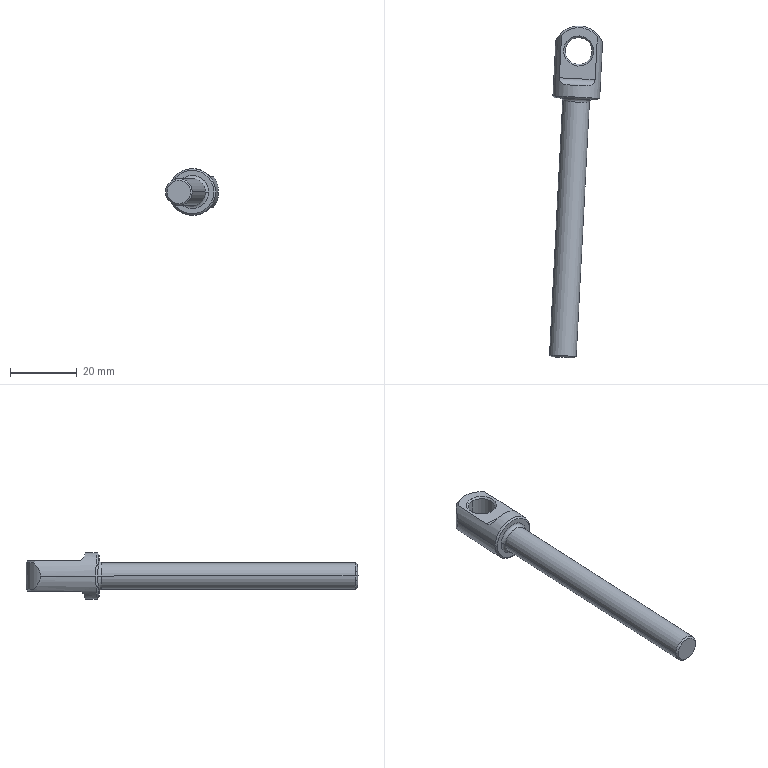Component | SolidWorks | CylinderAxis-1 | 1 solid | 28 faces | box 15.86 x 99.37 x 14 mm | volume 6011 mm3 | cone 11 | cylinder 9 | plane 6 | torus 2 | commonest cylinder face diameters 8 x4 14 x2 4 x2 15 x1
STEP:
#1=COLOUR_RGB('',0.7922,0.8196,0.9333);
#2=FILL_AREA_STYLE_COLOUR('',#1);
#3=FILL_AREA_STYLE('',(#2));
#4=SURFACE_STYLE_FILL_AREA(#3);
#5=SURFACE_SIDE_STYLE('',(#4));
#6=SURFACE_STYLE_USAGE(.BOTH.,#5);
#7=PRESENTATION_STYLE_ASSIGNMENT((#6));
#8=CARTESIAN_POINT('',(4.691,-4.191,6.691));
#9=VERTEX_POINT('',#8);
#10=CARTESIAN_POINT('',(4.415,-4.176,6.691));
#11=VERTEX_POINT('',#10);
#12=CARTESIAN_POINT('',(4.553,-4.184,6.691));
#13=DIRECTION('',(-0.0519,-0.9987,0.));
#14=DIRECTION('',(0.9987,-0.0519,0.));
#15=AXIS2_PLACEMENT_3D('',#12,#13,#14);
#16=CIRCLE('',#15,0.1378);
#17=EDGE_CURVE('',#9,#11,#16,.T.);
#18=ORIENTED_EDGE('',*,*,#17,.F.);
#19=CARTESIAN_POINT('',(4.711,-4.172,6.691));
#20=VERTEX_POINT('',#19);
#21=CARTESIAN_POINT('',(4.691,-4.191,6.691));
#22=DIRECTION('',(0.7429,0.6695,0.));
#23=VECTOR('',#22,39.37);
#24=LINE('',#21,#23);
#25=EDGE_CURVE('',#9,#20,#24,.T.);
#26=ORIENTED_EDGE('',*,*,#25,.T.);
#27=CARTESIAN_POINT('',(4.397,-4.156,6.691));
#28=VERTEX_POINT('',#27);
#29=CARTESIAN_POINT('',(4.554,-4.164,6.691));
#30=DIRECTION('',(0.0519,0.9987,-0.));
#31=DIRECTION('',(0.9987,-0.0519,0.));
#32=AXIS2_PLACEMENT_3D('',#29,#30,#31);
#33=CIRCLE('',#32,0.1575);
#34=EDGE_CURVE('',#28,#20,#33,.T.);
#35=ORIENTED_EDGE('',*,*,#34,.F.);
#36=CARTESIAN_POINT('',(4.415,-4.176,6.691));
#37=DIRECTION('',(-0.6695,0.7429,-0.));
#38=VECTOR('',#37,39.37);
#39=LINE('',#36,#38);
#40=EDGE_CURVE('',#11,#28,#39,.T.);
#41=ORIENTED_EDGE('',*,*,#40,.F.);
#42=EDGE_LOOP('',(#18,#26,#35,#41));
#43=FACE_OUTER_BOUND('',#42,.T.);
#44=CARTESIAN_POINT('',(4.553,-4.184,6.691));
#45=DIRECTION('',(0.0519,0.9987,-0.));
#46=DIRECTION('',(-0.9987,0.0519,0.));
#47=AXIS2_PLACEMENT_3D('',#44,#45,#46);
#48=CONICAL_SURFACE('',#47,0.1378,0.7854);
#49=ADVANCED_FACE('',(#43),#48,.T.);
#50=CARTESIAN_POINT('',(4.755,-0.2988,6.514));
#51=VERTEX_POINT('',#50);
#52=CARTESIAN_POINT('',(4.961,-0.408,6.514));
#53=VERTEX_POINT('',#52);
#54=CARTESIAN_POINT('',(4.741,-0.574,6.514));
#55=DIRECTION('',(0.,-0.,-1.));
#56=DIRECTION('',(0.0519,0.9987,0.));
#57=AXIS2_PLACEMENT_3D('',#54,#55,#56);
#58=CIRCLE('',#57,0.2756);
#59=EDGE_CURVE('',#51,#53,#58,.T.);
#60=ORIENTED_EDGE('',*,*,#59,.F.);
#61=CARTESIAN_POINT('',(4.756,-0.2791,6.534));
#62=VERTEX_POINT('',#61);
#63=CARTESIAN_POINT('',(4.755,-0.2988,6.514));
#64=DIRECTION('',(0.0367,0.7062,0.7071));
#65=VECTOR('',#64,39.37);
#66=LINE('',#63,#65);
#67=EDGE_CURVE('',#51,#62,#66,.T.);
#68=ORIENTED_EDGE('',*,*,#67,.T.);
#69=CARTESIAN_POINT('',(4.976,-0.3961,6.534));
#70=VERTEX_POINT('',#69);
#71=CARTESIAN_POINT('',(4.741,-0.574,6.534));
#72=DIRECTION('',(-0.,0.,1.));
#73=DIRECTION('',(0.0519,0.9987,0.));
#74=AXIS2_PLACEMENT_3D('',#71,#72,#73);
#75=CIRCLE('',#74,0.2953);
#76=EDGE_CURVE('',#70,#62,#75,.T.);
#77=ORIENTED_EDGE('',*,*,#76,.F.);
#78=CARTESIAN_POINT('',(4.961,-0.408,6.514));
#79=CARTESIAN_POINT('',(4.966,-0.4047,6.521));
#80=CARTESIAN_POINT('',(4.972,-0.4007,6.527));
#81=CARTESIAN_POINT('',(4.976,-0.3961,6.534));
#82=B_SPLINE_CURVE_WITH_KNOTS('',3,(#78,#79,#80,#81),.UNSPECIFIED.,.F.,.F.,(4,4),(0.,0.0007071),.UNSPECIFIED.);
#83=EDGE_CURVE('',#53,#70,#82,.T.);
#84=ORIENTED_EDGE('',*,*,#83,.F.);
#85=EDGE_LOOP('',(#60,#68,#77,#84));
#86=FACE_OUTER_BOUND('',#85,.T.);
#87=CARTESIAN_POINT('',(4.741,-0.574,6.514));
#88=DIRECTION('',(-0.,0.,1.));
#89=DIRECTION('',(0.0519,0.9987,0.));
#90=AXIS2_PLACEMENT_3D('',#87,#88,#89);
#91=CONICAL_SURFACE('',#90,0.2756,0.7854);
#92=ADVANCED_FACE('',(#86),#91,.T.);
#93=CARTESIAN_POINT('',(4.733,-0.7313,6.849));
#94=VERTEX_POINT('',#93);
#95=CARTESIAN_POINT('',(4.749,-0.4167,6.849));
#96=VERTEX_POINT('',#95);
#97=CARTESIAN_POINT('',(4.741,-0.574,6.849));
#98=DIRECTION('',(-0.,0.,1.));
#99=DIRECTION('',(-0.0519,-0.9987,0.));
#100=AXIS2_PLACEMENT_3D('',#97,#98,#99);
#101=CIRCLE('',#100,0.1575);
#102=EDGE_CURVE('',#94,#96,#101,.T.);
#103=ORIENTED_EDGE('',*,*,#102,.F.);
#104=CARTESIAN_POINT('',(4.732,-0.7509,6.869));
#105=VERTEX_POINT('',#104);
#106=CARTESIAN_POINT('',(4.732,-0.7509,6.869));
#107=DIRECTION('',(-0.0367,-0.7062,0.7071));
#108=VECTOR('',#107,39.37);
#109=LINE('',#106,#108);
#110=EDGE_CURVE('',#94,#105,#109,.T.);
#111=ORIENTED_EDGE('',*,*,#110,.T.);
#112=CARTESIAN_POINT('',(4.75,-0.3971,6.869));
#113=VERTEX_POINT('',#112);
#114=CARTESIAN_POINT('',(4.741,-0.574,6.869));
#115=DIRECTION('',(0.,-0.,-1.));
#116=DIRECTION('',(-0.0519,-0.9987,0.));
#117=AXIS2_PLACEMENT_3D('',#114,#115,#116);
#118=CIRCLE('',#117,0.1772);
#119=EDGE_CURVE('',#113,#105,#118,.T.);
#120=ORIENTED_EDGE('',*,*,#119,.F.);
#121=CARTESIAN_POINT('',(4.75,-0.3971,6.869));
#122=DIRECTION('',(0.0367,0.7062,0.7071));
#123=VECTOR('',#122,39.37);
#124=LINE('',#121,#123);
#125=EDGE_CURVE('',#96,#113,#124,.T.);
#126=ORIENTED_EDGE('',*,*,#125,.F.);
#127=EDGE_LOOP('',(#103,#111,#120,#126));
#128=FACE_OUTER_BOUND('',#127,.T.);
#129=CARTESIAN_POINT('',(4.741,-0.574,6.869));
#130=DIRECTION('',(-0.,0.,1.));
#131=DIRECTION('',(0.0519,0.9987,0.));
#132=AXIS2_PLACEMENT_3D('',#129,#130,#131);
#133=CONICAL_SURFACE('',#132,0.1772,0.7854);
#134=ADVANCED_FACE('',(#128),#133,.F.);
#135=CARTESIAN_POINT('',(4.749,-0.4167,6.534));
#136=VERTEX_POINT('',#135);
#137=CARTESIAN_POINT('',(4.733,-0.7313,6.534));
#138=VERTEX_POINT('',#137);
#139=CARTESIAN_POINT('',(4.741,-0.574,6.534));
#140=DIRECTION('',(0.,-0.,-1.));
#141=DIRECTION('',(0.0519,0.9987,0.));
#142=AXIS2_PLACEMENT_3D('',#139,#140,#141);
#143=CIRCLE('',#142,0.1575);
#144=EDGE_CURVE('',#136,#138,#143,.T.);
#145=ORIENTED_EDGE('',*,*,#144,.F.);
#146=CARTESIAN_POINT('',(4.75,-0.3971,6.514));
#147=VERTEX_POINT('',#146);
#148=CARTESIAN_POINT('',(4.75,-0.3971,6.514));
#149=DIRECTION('',(0.0367,0.7062,-0.7071));
#150=VECTOR('',#149,39.37);
#151=LINE('',#148,#150);
#152=EDGE_CURVE('',#136,#147,#151,.T.);
#153=ORIENTED_EDGE('',*,*,#152,.T.);
#154=CARTESIAN_POINT('',(4.732,-0.7509,6.514));
#155=VERTEX_POINT('',#154);
#156=CARTESIAN_POINT('',(4.741,-0.574,6.514));
#157=DIRECTION('',(-0.,0.,1.));
#158=DIRECTION('',(0.0519,0.9987,0.));
#159=AXIS2_PLACEMENT_3D('',#156,#157,#158);
#160=CIRCLE('',#159,0.1772);
#161=EDGE_CURVE('',#155,#147,#160,.T.);
#162=ORIENTED_EDGE('',*,*,#161,.F.);
#163=CARTESIAN_POINT('',(4.732,-0.7509,6.514));
#164=DIRECTION('',(-0.0367,-0.7062,-0.7071));
#165=VECTOR('',#164,39.37);
#166=LINE('',#163,#165);
#167=EDGE_CURVE('',#138,#155,#166,.T.);
#168=ORIENTED_EDGE('',*,*,#167,.F.);
#169=EDGE_LOOP('',(#145,#153,#162,#168));
#170=FACE_OUTER_BOUND('',#169,.T.);
#171=CARTESIAN_POINT('',(4.741,-0.574,6.514));
#172=DIRECTION('',(0.,-0.,-1.));
#173=DIRECTION('',(-0.0519,-0.9987,0.));
#174=AXIS2_PLACEMENT_3D('',#171,#172,#173);
#175=CONICAL_SURFACE('',#174,0.1772,0.7854);
#176=ADVANCED_FACE('',(#170),#175,.F.);
#177=CARTESIAN_POINT('',(4.908,-1.147,6.691));
#178=VERTEX_POINT('',#177);
#179=CARTESIAN_POINT('',(4.515,-1.126,6.691));
#180=VERTEX_POINT('',#179);
#181=CARTESIAN_POINT('',(4.711,-1.137,6.691));
#182=DIRECTION('',(0.0519,0.9987,-0.));
#183=DIRECTION('',(-0.9987,0.0519,0.));
#184=AXIS2_PLACEMENT_3D('',#181,#182,#183);
#185=CIRCLE('',#184,0.1969);
#186=EDGE_CURVE('',#178,#180,#185,.T.);
#187=ORIENTED_EDGE('',*,*,#186,.F.);
#188=CARTESIAN_POINT('',(4.867,-1.184,6.691));
#189=VERTEX_POINT('',#188);
#190=CARTESIAN_POINT('',(4.906,-1.186,6.691));
#191=DIRECTION('',(-0.,0.,1.));
#192=DIRECTION('',(1.,0.,0.));
#193=AXIS2_PLACEMENT_3D('',#190,#191,#192);
#194=CIRCLE('',#193,0.03937);
#195=EDGE_CURVE('',#178,#189,#194,.T.);
#196=ORIENTED_EDGE('',*,*,#195,.T.);
#197=CARTESIAN_POINT('',(4.552,-1.168,6.691));
#198=VERTEX_POINT('',#197);
#199=CARTESIAN_POINT('',(4.709,-1.176,6.691));
#200=DIRECTION('',(-0.0519,-0.9987,0.));
#201=DIRECTION('',(-0.9987,0.0519,0.));
#202=AXIS2_PLACEMENT_3D('',#199,#200,#201);
#203=CIRCLE('',#202,0.1575);
#204=EDGE_CURVE('',#198,#189,#203,.T.);
#205=ORIENTED_EDGE('',*,*,#204,.F.);
#206=CARTESIAN_POINT('',(4.513,-1.166,6.691));
#207=DIRECTION('',(0.,-0.,-1.));
#208=DIRECTION('',(0.,1.,0.));
#209=AXIS2_PLACEMENT_3D('',#206,#207,#208);
#210=CIRCLE('',#209,0.03937);
#211=EDGE_CURVE('',#180,#198,#210,.T.);
#212=ORIENTED_EDGE('',*,*,#211,.F.);
#213=EDGE_LOOP('',(#187,#196,#205,#212));
#214=FACE_OUTER_BOUND('',#213,.T.);
#215=CARTESIAN_POINT('',(4.709,-1.176,6.691));
#216=DIRECTION('',(0.0519,0.9987,-0.));
#217=DIRECTION('',(-0.9987,0.0519,-0.));
#218=AXIS2_PLACEMENT_3D('',#215,#216,#217);
#219=TOROIDAL_SURFACE('',#218,0.1969,0.03937);
#220=ADVANCED_FACE('',(#214),#219,.F.);
#221=CARTESIAN_POINT('',(4.967,-1.15,6.691));
#222=VERTEX_POINT('',#221);
#223=CARTESIAN_POINT('',(4.456,-1.123,6.691));
#224=VERTEX_POINT('',#223);
#225=CARTESIAN_POINT('',(4.711,-1.137,6.691));
#226=DIRECTION('',(-0.0519,-0.9987,0.));
#227=DIRECTION('',(-0.9987,0.0519,0.));
#228=AXIS2_PLACEMENT_3D('',#225,#226,#227);
#229=CIRCLE('',#228,0.2559);
#230=EDGE_CURVE('',#222,#224,#229,.T.);
#231=ORIENTED_EDGE('',*,*,#230,.F.);
#232=CARTESIAN_POINT('',(4.988,-1.131,6.691));
#233=VERTEX_POINT('',#232);
#234=CARTESIAN_POINT('',(4.988,-1.131,6.691));
#235=DIRECTION('',(0.7429,0.6695,0.));
#236=VECTOR('',#235,39.37);
#237=LINE('',#234,#236);
#238=EDGE_CURVE('',#222,#233,#237,.T.);
#239=ORIENTED_EDGE('',*,*,#238,.T.);
#240=CARTESIAN_POINT('',(4.437,-1.103,6.691));
#241=VERTEX_POINT('',#240);
#242=CARTESIAN_POINT('',(4.712,-1.117,6.691));
#243=DIRECTION('',(0.0519,0.9987,-0.));
#244=DIRECTION('',(-0.9987,0.0519,0.));
#245=AXIS2_PLACEMENT_3D('',#242,#243,#244);
#246=CIRCLE('',#245,0.2756);
#247=EDGE_CURVE('',#241,#233,#246,.T.);
#248=ORIENTED_EDGE('',*,*,#247,.F.);
#249=CARTESIAN_POINT('',(4.437,-1.103,6.691));
#250=DIRECTION('',(-0.6695,0.7429,-0.));
#251=VECTOR('',#250,39.37);
#252=LINE('',#249,#251);
#253=EDGE_CURVE('',#224,#241,#252,.T.);
#254=ORIENTED_EDGE('',*,*,#253,.F.);
#255=EDGE_LOOP('',(#231,#239,#248,#254));
#256=FACE_OUTER_BOUND('',#255,.T.);
#257=CARTESIAN_POINT('',(4.712,-1.117,6.691));
#258=DIRECTION('',(0.0519,0.9987,-0.));
#259=DIRECTION('',(-0.9987,0.0519,0.));
#260=AXIS2_PLACEMENT_3D('',#257,#258,#259);
#261=CONICAL_SURFACE('',#260,0.2756,0.7854);
#262=ADVANCED_FACE('',(#256),#261,.T.);
#263=ORIENTED_EDGE('',*,*,#34,.T.);
#264=CARTESIAN_POINT('',(4.71,-4.192,6.691));
#265=DIRECTION('',(0.0519,0.9987,-0.));
#266=VECTOR('',#265,39.37);
#267=LINE('',#264,#266);
#268=EDGE_CURVE('',#20,#189,#267,.T.);
#269=ORIENTED_EDGE('',*,*,#268,.T.);
#270=CARTESIAN_POINT('',(4.709,-1.176,6.691));
#271=DIRECTION('',(-0.0519,-0.9987,0.));
#272=DIRECTION('',(-0.9987,0.0519,0.));
#273=AXIS2_PLACEMENT_3D('',#270,#271,#272);
#274=CIRCLE('',#273,0.1575);
#275=EDGE_CURVE('',#189,#198,#274,.T.);
#276=ORIENTED_EDGE('',*,*,#275,.T.);
#277=CARTESIAN_POINT('',(4.396,-4.175,6.691));
#278=DIRECTION('',(0.0519,0.9987,-0.));
#279=VECTOR('',#278,39.37);
#280=LINE('',#277,#279);
#281=EDGE_CURVE('',#28,#198,#280,.T.);
#282=ORIENTED_EDGE('',*,*,#281,.F.);
#283=EDGE_LOOP('',(#263,#269,#276,#282));
#284=FACE_OUTER_BOUND('',#283,.T.);
#285=CARTESIAN_POINT('',(4.553,-4.184,6.691));
#286=DIRECTION('',(0.0519,0.9987,-0.));
#287=DIRECTION('',(-0.9987,0.0519,0.));
#288=AXIS2_PLACEMENT_3D('',#285,#286,#287);
#289=CYLINDRICAL_SURFACE('',#288,0.1575);
#290=ADVANCED_FACE('',(#284),#289,.T.);
#291=ORIENTED_EDGE('',*,*,#144,.T.);
#292=CARTESIAN_POINT('',(4.733,-0.7313,6.199));
#293=DIRECTION('',(-0.,0.,1.));
#294=VECTOR('',#293,39.37);
#295=LINE('',#292,#294);
#296=EDGE_CURVE('',#138,#94,#295,.T.);
#297=ORIENTED_EDGE('',*,*,#296,.T.);
#298=ORIENTED_EDGE('',*,*,#102,.T.);
#299=CARTESIAN_POINT('',(4.749,-0.4167,6.199));
#300=DIRECTION('',(-0.,0.,1.));
#301=VECTOR('',#300,39.37);
#302=LINE('',#299,#301);
#303=EDGE_CURVE('',#136,#96,#302,.T.);
#304=ORIENTED_EDGE('',*,*,#303,.F.);
#305=EDGE_LOOP('',(#291,#297,#298,#304));
#306=FACE_OUTER_BOUND('',#305,.T.);
#307=CARTESIAN_POINT('',(4.741,-0.574,6.199));
#308=DIRECTION('',(-0.,0.,1.));
#309=DIRECTION('',(0.0519,0.9987,0.));
#310=AXIS2_PLACEMENT_3D('',#307,#308,#309);
#311=CYLINDRICAL_SURFACE('',#310,0.1575);
#312=ADVANCED_FACE('',(#306),#311,.F.);
#313=CARTESIAN_POINT('',(4.525,-0.3727,6.849));
#314=VERTEX_POINT('',#313);
#315=CARTESIAN_POINT('',(4.471,-0.4538,6.691));
#316=VERTEX_POINT('',#315);
#317=CARTESIAN_POINT('',(4.525,-0.3727,6.849));
#318=CARTESIAN_POINT('',(4.517,-0.3812,6.838));
#319=CARTESIAN_POINT('',(4.51,-0.3897,6.827));
#320=CARTESIAN_POINT('',(4.497,-0.4067,6.804));
#321=CARTESIAN_POINT('',(4.492,-0.4152,6.792));
#322=CARTESIAN_POINT('',(4.482,-0.4311,6.766));
#323=CARTESIAN_POINT('',(4.478,-0.4386,6.752));
#324=CARTESIAN_POINT('',(4.474,-0.4472,6.73));
#325=CARTESIAN_POINT('',(4.473,-0.4496,6.723));
#326=CARTESIAN_POINT('',(4.471,-0.4529,6.707));
#327=CARTESIAN_POINT('',(4.471,-0.4538,6.699));
#328=CARTESIAN_POINT('',(4.471,-0.4538,6.691));
#329=B_SPLINE_CURVE_WITH_KNOTS('',3,(#317,#318,#319,#320,#321,#322,#323,#324,#325,#326,#327,#328),.UNSPECIFIED.,.F.,.F.,(4,2,2,2,2,4),(0.0007506,0.001947,0.003143,0.004339,0.004937,0.005535),.UNSPECIFIED.);
#330=EDGE_CURVE('',#314,#316,#329,.T.);
#331=ORIENTED_EDGE('',*,*,#330,.T.);
#332=CARTESIAN_POINT('',(4.444,-0.9649,6.691));
#333=DIRECTION('',(-0.0519,-0.9987,0.));
#334=VECTOR('',#333,39.37);
#335=LINE('',#332,#334);
#336=EDGE_CURVE('',#316,#241,#335,.T.);
#337=ORIENTED_EDGE('',*,*,#336,.T.);
#338=ORIENTED_EDGE('',*,*,#247,.T.);
#339=CARTESIAN_POINT('',(5.021,-0.4824,6.691));
#340=VERTEX_POINT('',#339);
#341=CARTESIAN_POINT('',(4.995,-0.9935,6.691));
#342=DIRECTION('',(-0.0519,-0.9987,0.));
#343=VECTOR('',#342,39.37);
#344=LINE('',#341,#343);
#345=EDGE_CURVE('',#340,#233,#344,.T.);
#346=ORIENTED_EDGE('',*,*,#345,.F.);
#347=CARTESIAN_POINT('',(4.976,-0.3961,6.849));
#348=VERTEX_POINT('',#347);
#349=CARTESIAN_POINT('',(5.021,-0.4824,6.691));
#350=CARTESIAN_POINT('',(5.021,-0.4824,6.699));
#351=CARTESIAN_POINT('',(5.021,-0.4815,6.707));
#352=CARTESIAN_POINT('',(5.02,-0.4781,6.723));
#353=CARTESIAN_POINT('',(5.019,-0.4755,6.73));
#354=CARTESIAN_POINT('',(5.016,-0.4666,6.752));
#355=CARTESIAN_POINT('',(5.013,-0.4589,6.766));
#356=CARTESIAN_POINT('',(5.005,-0.442,6.792));
#357=CARTESIAN_POINT('',(5.,-0.433,6.804));
#358=CARTESIAN_POINT('',(4.99,-0.4147,6.827));
#359=CARTESIAN_POINT('',(4.983,-0.4054,6.838));
#360=CARTESIAN_POINT('',(4.976,-0.3961,6.849));
#361=B_SPLINE_CURVE_WITH_KNOTS('',3,(#349,#350,#351,#352,#353,#354,#355,#356,#357,#358,#359,#360),.UNSPECIFIED.,.F.,.F.,(4,2,2,2,2,4),(0.005535,0.006132,0.006728,0.007922,0.009116,0.01031),.UNSPECIFIED.);
#362=EDGE_CURVE('',#340,#348,#361,.T.);
#363=ORIENTED_EDGE('',*,*,#362,.T.);
#364=CARTESIAN_POINT('',(4.961,-0.408,6.869));
#365=VERTEX_POINT('',#364);
#366=CARTESIAN_POINT('',(4.976,-0.3961,6.849));
#367=CARTESIAN_POINT('',(4.972,-0.4007,6.855));
#368=CARTESIAN_POINT('',(4.966,-0.4047,6.862));
#369=CARTESIAN_POINT('',(4.961,-0.408,6.869));
#370=B_SPLINE_CURVE_WITH_KNOTS('',3,(#366,#367,#368,#369),.UNSPECIFIED.,.F.,.F.,(4,4),(0.,0.0007071),.UNSPECIFIED.);
#371=EDGE_CURVE('',#348,#365,#370,.T.);
#372=ORIENTED_EDGE('',*,*,#371,.T.);
#373=CARTESIAN_POINT('',(4.935,-0.9116,6.869));
#374=VERTEX_POINT('',#373);
#375=CARTESIAN_POINT('',(4.957,-0.4791,6.869));
#376=DIRECTION('',(-0.0519,-0.9987,0.));
#377=VECTOR('',#376,39.37);
#378=LINE('',#375,#377);
#379=EDGE_CURVE('',#365,#374,#378,.T.);
#380=ORIENTED_EDGE('',*,*,#379,.T.);
#381=CARTESIAN_POINT('',(4.822,-0.9846,6.947));
#382=VERTEX_POINT('',#381);
#383=CARTESIAN_POINT('',(4.935,-0.9116,6.869));
#384=CARTESIAN_POINT('',(4.934,-0.9189,6.869));
#385=CARTESIAN_POINT('',(4.933,-0.926,6.87));
#386=CARTESIAN_POINT('',(4.929,-0.9396,6.874));
#387=CARTESIAN_POINT('',(4.926,-0.9458,6.876));
#388=CARTESIAN_POINT('',(4.919,-0.9568,6.883));
#389=CARTESIAN_POINT('',(4.915,-0.9615,6.887));
#390=CARTESIAN_POINT('',(4.906,-0.9695,6.895));
#391=CARTESIAN_POINT('',(4.901,-0.9727,6.9));
#392=CARTESIAN_POINT('',(4.89,-0.9778,6.908));
#393=CARTESIAN_POINT('',(4.885,-0.9797,6.912));
#394=CARTESIAN_POINT('',(4.873,-0.9826,6.92));
#395=CARTESIAN_POINT('',(4.867,-0.9836,6.924));
#396=CARTESIAN_POINT('',(4.848,-0.9854,6.935));
#397=CARTESIAN_POINT('',(4.835,-0.9853,6.942));
#398=CARTESIAN_POINT('',(4.822,-0.9846,6.947));
#399=B_SPLINE_CURVE_WITH_KNOTS('',3,(#383,#384,#385,#386,#387,#388,#389,#390,#391,#392,#393,#394,#395,#396,#397,#398),.UNSPECIFIED.,.F.,.F.,(4,2,2,2,2,2,2,4),(0.,0.0005534,0.001107,0.00166,0.002213,0.002767,0.00332,0.004427),.UNSPECIFIED.);
#400=EDGE_CURVE('',#374,#382,#399,.T.);
#401=ORIENTED_EDGE('',*,*,#400,.T.);
#402=CARTESIAN_POINT('',(4.617,-0.9739,6.947));
#403=VERTEX_POINT('',#402);
#404=CARTESIAN_POINT('',(4.72,-0.9792,6.691));
#405=DIRECTION('',(0.0519,0.9987,-0.));
#406=DIRECTION('',(-0.9987,0.0519,0.));
#407=AXIS2_PLACEMENT_3D('',#404,#405,#406);
#408=CIRCLE('',#407,0.2756);
#409=EDGE_CURVE('',#403,#382,#408,.T.);
#410=ORIENTED_EDGE('',*,*,#409,.F.);
#411=CARTESIAN_POINT('',(4.513,-0.8897,6.869));
#412=VERTEX_POINT('',#411);
#413=CARTESIAN_POINT('',(4.617,-0.9739,6.947));
#414=CARTESIAN_POINT('',(4.604,-0.9732,6.942));
#415=CARTESIAN_POINT('',(4.591,-0.972,6.936));
#416=CARTESIAN_POINT('',(4.573,-0.9683,6.925));
#417=CARTESIAN_POINT('',(4.567,-0.9668,6.921));
#418=CARTESIAN_POINT('',(4.556,-0.9628,6.913));
#419=CARTESIAN_POINT('',(4.55,-0.9602,6.908));
#420=CARTESIAN_POINT('',(4.54,-0.9541,6.9));
#421=CARTESIAN_POINT('',(4.535,-0.9503,6.895));
#422=CARTESIAN_POINT('',(4.527,-0.9415,6.887));
#423=CARTESIAN_POINT('',(4.524,-0.9365,6.883));
#424=CARTESIAN_POINT('',(4.518,-0.9248,6.876));
#425=CARTESIAN_POINT('',(4.516,-0.9183,6.874));
#426=CARTESIAN_POINT('',(4.513,-0.9044,6.87));
#427=CARTESIAN_POINT('',(4.513,-0.8971,6.869));
#428=CARTESIAN_POINT('',(4.513,-0.8897,6.869));
#429=B_SPLINE_CURVE_WITH_KNOTS('',3,(#413,#414,#415,#416,#417,#418,#419,#420,#421,#422,#423,#424,#425,#426,#427,#428),.UNSPECIFIED.,.F.,.F.,(4,2,2,2,2,2,2,4),(0.,0.001095,0.001642,0.002189,0.002736,0.003284,0.003831,0.004378),.UNSPECIFIED.);
#430=EDGE_CURVE('',#403,#412,#429,.T.);
#431=ORIENTED_EDGE('',*,*,#430,.T.);
#432=CARTESIAN_POINT('',(4.539,-0.3861,6.869));
#433=VERTEX_POINT('',#432);
#434=CARTESIAN_POINT('',(4.535,-0.4572,6.869));
#435=DIRECTION('',(-0.0519,-0.9987,0.));
#436=VECTOR('',#435,39.37);
#437=LINE('',#434,#436);
#438=EDGE_CURVE('',#433,#412,#437,.T.);
#439=ORIENTED_EDGE('',*,*,#438,.F.);
#440=CARTESIAN_POINT('',(4.539,-0.3861,6.869));
#441=CARTESIAN_POINT('',(4.534,-0.3822,6.862));
#442=CARTESIAN_POINT('',(4.529,-0.3777,6.855));
#443=CARTESIAN_POINT('',(4.525,-0.3727,6.849));
#444=B_SPLINE_CURVE_WITH_KNOTS('',3,(#440,#441,#442,#443),.UNSPECIFIED.,.F.,.F.,(4,4),(0.,0.0007071),.UNSPECIFIED.);
#445=EDGE_CURVE('',#433,#314,#444,.T.);
#446=ORIENTED_EDGE('',*,*,#445,.T.);
#447=EDGE_LOOP('',(#331,#337,#338,#346,#363,#372,#380,#401,#410,#431,#439,#446));
#448=FACE_OUTER_BOUND('',#447,.T.);
#449=CARTESIAN_POINT('',(4.72,-0.9792,6.691));
#450=DIRECTION('',(-0.0519,-0.9987,0.));
#451=DIRECTION('',(0.9987,-0.0519,0.));
#452=AXIS2_PLACEMENT_3D('',#449,#450,#451);
#453=CYLINDRICAL_SURFACE('',#452,0.2756);
#454=ADVANCED_FACE('',(#448),#453,.T.);
#455=CARTESIAN_POINT('',(4.711,-1.137,6.691));
#456=DIRECTION('',(0.0519,0.9987,-0.));
#457=DIRECTION('',(-0.9987,0.0519,0.));
#458=AXIS2_PLACEMENT_3D('',#455,#456,#457);
#459=CIRCLE('',#458,0.1969);
#460=EDGE_CURVE('',#180,#178,#459,.T.);
#461=ORIENTED_EDGE('',*,*,#460,.T.);
#462=ORIENTED_EDGE('',*,*,#186,.T.);
#463=EDGE_LOOP('',(#461,#462));
#464=FACE_BOUND('',#463,.T.);
#465=CARTESIAN_POINT('',(4.711,-1.137,6.691));
#466=DIRECTION('',(-0.0519,-0.9987,0.));
#467=DIRECTION('',(-0.9987,0.0519,0.));
#468=AXIS2_PLACEMENT_3D('',#465,#466,#467);
#469=CIRCLE('',#468,0.2559);
#470=EDGE_CURVE('',#224,#222,#469,.T.);
#471=ORIENTED_EDGE('',*,*,#470,.T.);
#472=ORIENTED_EDGE('',*,*,#230,.T.);
#473=EDGE_LOOP('',(#471,#472));
#474=FACE_OUTER_BOUND('',#473,.T.);
#475=CARTESIAN_POINT('',(4.711,-1.137,6.691));
#476=DIRECTION('',(0.0519,0.9987,-0.));
#477=DIRECTION('',(-0.9987,0.0519,-0.));
#478=AXIS2_PLACEMENT_3D('',#475,#476,#477);
#479=PLANE('',#478);
#480=ADVANCED_FACE('',(#464,#474),#479,.F.);
#481=ORIENTED_EDGE('',*,*,#409,.T.);
#482=CARTESIAN_POINT('',(4.72,-0.9792,6.947));
#483=DIRECTION('',(-0.9987,0.0519,-0.));
#484=VECTOR('',#483,39.37);
#485=LINE('',#482,#484);
#486=EDGE_CURVE('',#382,#403,#485,.T.);
#487=ORIENTED_EDGE('',*,*,#486,.T.);
#488=EDGE_LOOP('',(#481,#487));
#489=FACE_OUTER_BOUND('',#488,.T.);
#490=CARTESIAN_POINT('',(4.72,-0.9792,6.691));
#491=DIRECTION('',(0.0519,0.9987,-0.));
#492=DIRECTION('',(-0.9987,0.0519,-0.));
#493=AXIS2_PLACEMENT_3D('',#490,#491,#492);
#494=PLANE('',#493);
#495=ADVANCED_FACE('',(#489),#494,.T.);
#496=ORIENTED_EDGE('',*,*,#336,.F.);
#497=CARTESIAN_POINT('',(4.525,-0.3727,6.534));
#498=VERTEX_POINT('',#497);
#499=CARTESIAN_POINT('',(4.471,-0.4538,6.691));
#500=CARTESIAN_POINT('',(4.471,-0.4538,6.683));
#501=CARTESIAN_POINT('',(4.471,-0.4529,6.675));
#502=CARTESIAN_POINT('',(4.473,-0.4496,6.66));
#503=CARTESIAN_POINT('',(4.474,-0.4472,6.652));
#504=CARTESIAN_POINT('',(4.478,-0.4387,6.631));
#505=CARTESIAN_POINT('',(4.482,-0.4313,6.617));
#506=CARTESIAN_POINT('',(4.492,-0.4153,6.591));
#507=CARTESIAN_POINT('',(4.497,-0.4068,6.579));
#508=CARTESIAN_POINT('',(4.51,-0.3898,6.556));
#509=CARTESIAN_POINT('',(4.517,-0.3812,6.545));
#510=CARTESIAN_POINT('',(4.525,-0.3727,6.534));
#511=B_SPLINE_CURVE_WITH_KNOTS('',3,(#499,#500,#501,#502,#503,#504,#505,#506,#507,#508,#509,#510),.UNSPECIFIED.,.F.,.F.,(4,2,2,2,2,4),(0.005535,0.006132,0.006728,0.007922,0.009116,0.01031),.UNSPECIFIED.);
#512=EDGE_CURVE('',#316,#498,#511,.T.);
#513=ORIENTED_EDGE('',*,*,#512,.T.);
#514=CARTESIAN_POINT('',(4.539,-0.3861,6.514));
#515=VERTEX_POINT('',#514);
#516=CARTESIAN_POINT('',(4.525,-0.3727,6.534));
#517=CARTESIAN_POINT('',(4.529,-0.3777,6.527));
#518=CARTESIAN_POINT('',(4.534,-0.3822,6.521));
#519=CARTESIAN_POINT('',(4.539,-0.3861,6.514));
#520=B_SPLINE_CURVE_WITH_KNOTS('',3,(#516,#517,#518,#519),.UNSPECIFIED.,.F.,.F.,(4,4),(0.,0.0007071),.UNSPECIFIED.);
#521=EDGE_CURVE('',#498,#515,#520,.T.);
#522=ORIENTED_EDGE('',*,*,#521,.T.);
#523=CARTESIAN_POINT('',(4.513,-0.8897,6.514));
#524=VERTEX_POINT('',#523);
#525=CARTESIAN_POINT('',(4.535,-0.4572,6.514));
#526=DIRECTION('',(-0.0519,-0.9987,0.));
#527=VECTOR('',#526,39.37);
#528=LINE('',#525,#527);
#529=EDGE_CURVE('',#515,#524,#528,.T.);
#530=ORIENTED_EDGE('',*,*,#529,.T.);
#531=CARTESIAN_POINT('',(4.617,-0.9739,6.436));
#532=VERTEX_POINT('',#531);
#533=CARTESIAN_POINT('',(4.513,-0.8897,6.514));
#534=CARTESIAN_POINT('',(4.513,-0.897,6.514));
#535=CARTESIAN_POINT('',(4.513,-0.9042,6.513));
#536=CARTESIAN_POINT('',(4.516,-0.9182,6.509));
#537=CARTESIAN_POINT('',(4.518,-0.9246,6.507));
#538=CARTESIAN_POINT('',(4.524,-0.9363,6.5));
#539=CARTESIAN_POINT('',(4.527,-0.9414,6.496));
#540=CARTESIAN_POINT('',(4.535,-0.9503,6.488));
#541=CARTESIAN_POINT('',(4.54,-0.9539,6.483));
#542=CARTESIAN_POINT('',(4.55,-0.9601,6.475));
#543=CARTESIAN_POINT('',(4.555,-0.9626,6.471));
#544=CARTESIAN_POINT('',(4.567,-0.9667,6.462));
#545=CARTESIAN_POINT('',(4.573,-0.9683,6.459));
#546=CARTESIAN_POINT('',(4.591,-0.972,6.447));
#547=CARTESIAN_POINT('',(4.604,-0.9732,6.441));
#548=CARTESIAN_POINT('',(4.617,-0.9739,6.436));
#549=B_SPLINE_CURVE_WITH_KNOTS('',3,(#533,#534,#535,#536,#537,#538,#539,#540,#541,#542,#543,#544,#545,#546,#547,#548),.UNSPECIFIED.,.F.,.F.,(4,2,2,2,2,2,2,4),(0.,0.0005534,0.001107,0.00166,0.002213,0.002767,0.00332,0.004427),.UNSPECIFIED.);
#550=EDGE_CURVE('',#524,#532,#549,.T.);
#551=ORIENTED_EDGE('',*,*,#550,.T.);
#552=CARTESIAN_POINT('',(4.822,-0.9846,6.436));
#553=VERTEX_POINT('',#552);
#554=CARTESIAN_POINT('',(4.72,-0.9792,6.691));
#555=DIRECTION('',(0.0519,0.9987,-0.));
#556=DIRECTION('',(-0.9987,0.0519,0.));
#557=AXIS2_PLACEMENT_3D('',#554,#555,#556);
#558=CIRCLE('',#557,0.2756);
#559=EDGE_CURVE('',#553,#532,#558,.T.);
#560=ORIENTED_EDGE('',*,*,#559,.F.);
#561=CARTESIAN_POINT('',(4.935,-0.9116,6.514));
#562=VERTEX_POINT('',#561);
#563=CARTESIAN_POINT('',(4.822,-0.9846,6.436));
#564=CARTESIAN_POINT('',(4.835,-0.9853,6.441));
#565=CARTESIAN_POINT('',(4.848,-0.9854,6.447));
#566=CARTESIAN_POINT('',(4.867,-0.9836,6.458));
#567=CARTESIAN_POINT('',(4.873,-0.9827,6.462));
#568=CARTESIAN_POINT('',(4.884,-0.9798,6.47));
#569=CARTESIAN_POINT('',(4.89,-0.9779,6.475));
#570=CARTESIAN_POINT('',(4.901,-0.9728,6.483));
#571=CARTESIAN_POINT('',(4.906,-0.9696,6.488));
#572=CARTESIAN_POINT('',(4.915,-0.9617,6.496));
#573=CARTESIAN_POINT('',(4.919,-0.957,6.5));
#574=CARTESIAN_POINT('',(4.926,-0.946,6.506));
#575=CARTESIAN_POINT('',(4.929,-0.9398,6.509));
#576=CARTESIAN_POINT('',(4.933,-0.9262,6.513));
#577=CARTESIAN_POINT('',(4.934,-0.919,6.514));
#578=CARTESIAN_POINT('',(4.935,-0.9116,6.514));
#579=B_SPLINE_CURVE_WITH_KNOTS('',3,(#563,#564,#565,#566,#567,#568,#569,#570,#571,#572,#573,#574,#575,#576,#577,#578),.UNSPECIFIED.,.F.,.F.,(4,2,2,2,2,2,2,4),(0.,0.001095,0.001642,0.002189,0.002736,0.003284,0.003831,0.004378),.UNSPECIFIED.);
#580=EDGE_CURVE('',#553,#562,#579,.T.);
#581=ORIENTED_EDGE('',*,*,#580,.T.);
#582=CARTESIAN_POINT('',(4.957,-0.4791,6.514));
#583=DIRECTION('',(-0.0519,-0.9987,0.));
#584=VECTOR('',#583,39.37);
#585=LINE('',#582,#584);
#586=EDGE_CURVE('',#53,#562,#585,.T.);
#587=ORIENTED_EDGE('',*,*,#586,.F.);
#588=ORIENTED_EDGE('',*,*,#83,.T.);
#589=CARTESIAN_POINT('',(4.976,-0.3961,6.534));
#590=CARTESIAN_POINT('',(4.983,-0.4054,6.545));
#591=CARTESIAN_POINT('',(4.99,-0.4147,6.556));
#592=CARTESIAN_POINT('',(5.,-0.4329,6.579));
#593=CARTESIAN_POINT('',(5.005,-0.4419,6.591));
#594=CARTESIAN_POINT('',(5.013,-0.4587,6.617));
#595=CARTESIAN_POINT('',(5.016,-0.4666,6.63));
#596=CARTESIAN_POINT('',(5.019,-0.4755,6.652));
#597=CARTESIAN_POINT('',(5.02,-0.478,6.66));
#598=CARTESIAN_POINT('',(5.021,-0.4815,6.676));
#599=CARTESIAN_POINT('',(5.021,-0.4824,6.683));
#600=CARTESIAN_POINT('',(5.021,-0.4824,6.691));
#601=B_SPLINE_CURVE_WITH_KNOTS('',3,(#589,#590,#591,#592,#593,#594,#595,#596,#597,#598,#599,#600),.UNSPECIFIED.,.F.,.F.,(4,2,2,2,2,4),(0.0007506,0.001947,0.003143,0.004339,0.004937,0.005535),.UNSPECIFIED.);
#602=EDGE_CURVE('',#70,#340,#601,.T.);
#603=ORIENTED_EDGE('',*,*,#602,.T.);
#604=ORIENTED_EDGE('',*,*,#345,.T.);
#605=CARTESIAN_POINT('',(4.712,-1.117,6.691));
#606=DIRECTION('',(0.0519,0.9987,-0.));
#607=DIRECTION('',(-0.9987,0.0519,0.));
#608=AXIS2_PLACEMENT_3D('',#605,#606,#607);
#609=CIRCLE('',#608,0.2756);
#610=EDGE_CURVE('',#233,#241,#609,.T.);
#611=ORIENTED_EDGE('',*,*,#610,.T.);
#612=EDGE_LOOP('',(#496,#513,#522,#530,#551,#560,#581,#587,#588,#603,#604,#611));
#613=FACE_OUTER_BOUND('',#612,.T.);
#614=CARTESIAN_POINT('',(4.72,-0.9792,6.691));
#615=DIRECTION('',(-0.0519,-0.9987,0.));
#616=DIRECTION('',(0.9987,-0.0519,0.));
#617=AXIS2_PLACEMENT_3D('',#614,#615,#616);
#618=CYLINDRICAL_SURFACE('',#617,0.2756);
#619=ADVANCED_FACE('',(#613),#618,.T.);
#620=ORIENTED_EDGE('',*,*,#559,.T.);
#621=CARTESIAN_POINT('',(4.72,-0.9792,6.436));
#622=DIRECTION('',(0.9987,-0.0519,0.));
#623=VECTOR('',#622,39.37);
#624=LINE('',#621,#623);
#625=EDGE_CURVE('',#532,#553,#624,.T.);
#626=ORIENTED_EDGE('',*,*,#625,.T.);
#627=EDGE_LOOP('',(#620,#626));
#628=FACE_OUTER_BOUND('',#627,.T.);
#629=CARTESIAN_POINT('',(4.72,-0.9792,6.691));
#630=DIRECTION('',(0.0519,0.9987,-0.));
#631=DIRECTION('',(-0.9987,0.0519,-0.));
#632=AXIS2_PLACEMENT_3D('',#629,#630,#631);
#633=PLANE('',#632);
#634=ADVANCED_FACE('',(#628),#633,.T.);
#635=ORIENTED_EDGE('',*,*,#161,.T.);
#636=CARTESIAN_POINT('',(4.741,-0.574,6.514));
#637=DIRECTION('',(-0.,0.,1.));
#638=DIRECTION('',(0.0519,0.9987,0.));
#639=AXIS2_PLACEMENT_3D('',#636,#637,#638);
#640=CIRCLE('',#639,0.1772);
#641=EDGE_CURVE('',#147,#155,#640,.T.);
#642=ORIENTED_EDGE('',*,*,#641,.T.);
#643=EDGE_LOOP('',(#635,#642));
#644=FACE_BOUND('',#643,.T.);
#645=ORIENTED_EDGE('',*,*,#529,.F.);
#646=CARTESIAN_POINT('',(4.741,-0.574,6.514));
#647=DIRECTION('',(0.,-0.,-1.));
#648=DIRECTION('',(0.0519,0.9987,0.));
#649=AXIS2_PLACEMENT_3D('',#646,#647,#648);
#650=CIRCLE('',#649,0.2756);
#651=EDGE_CURVE('',#515,#51,#650,.T.);
#652=ORIENTED_EDGE('',*,*,#651,.T.);
#653=ORIENTED_EDGE('',*,*,#59,.T.);
#654=ORIENTED_EDGE('',*,*,#586,.T.);
#655=CARTESIAN_POINT('',(4.935,-0.9116,6.514));
#656=DIRECTION('',(-0.9987,0.0519,-0.));
#657=VECTOR('',#656,39.37);
#658=LINE('',#655,#657);
#659=EDGE_CURVE('',#562,#524,#658,.T.);
#660=ORIENTED_EDGE('',*,*,#659,.T.);
#661=EDGE_LOOP('',(#645,#652,#653,#654,#660));
#662=FACE_OUTER_BOUND('',#661,.T.);
#663=CARTESIAN_POINT('',(4.957,-0.4791,6.514));
#664=DIRECTION('',(-0.,0.,1.));
#665=DIRECTION('',(0.0519,0.9987,-0.));
#666=AXIS2_PLACEMENT_3D('',#663,#664,#665);
#667=PLANE('',#666);
#668=ADVANCED_FACE('',(#644,#662),#667,.F.);
#669=ORIENTED_EDGE('',*,*,#119,.T.);
#670=CARTESIAN_POINT('',(4.741,-0.574,6.869));
#671=DIRECTION('',(0.,-0.,-1.));
#672=DIRECTION('',(-0.0519,-0.9987,0.));
#673=AXIS2_PLACEMENT_3D('',#670,#671,#672);
#674=CIRCLE('',#673,0.1772);
#675=EDGE_CURVE('',#105,#113,#674,.T.);
#676=ORIENTED_EDGE('',*,*,#675,.T.);
#677=EDGE_LOOP('',(#669,#676));
#678=FACE_BOUND('',#677,.T.);
#679=ORIENTED_EDGE('',*,*,#379,.F.);
#680=CARTESIAN_POINT('',(4.741,-0.574,6.869));
#681=DIRECTION('',(-0.,0.,1.));
#682=DIRECTION('',(-0.0519,-0.9987,0.));
#683=AXIS2_PLACEMENT_3D('',#680,#681,#682);
#684=CIRCLE('',#683,0.2756);
#685=EDGE_CURVE('',#365,#433,#684,.T.);
#686=ORIENTED_EDGE('',*,*,#685,.T.);
#687=ORIENTED_EDGE('',*,*,#438,.T.);
#688=CARTESIAN_POINT('',(4.935,-0.9116,6.869));
#689=DIRECTION('',(0.9987,-0.0519,0.));
#690=VECTOR('',#689,39.37);
#691=LINE('',#688,#690);
#692=EDGE_CURVE('',#412,#374,#691,.T.);
#693=ORIENTED_EDGE('',*,*,#692,.T.);
#694=EDGE_LOOP('',(#679,#686,#687,#693));
#695=FACE_OUTER_BOUND('',#694,.T.);
#696=CARTESIAN_POINT('',(4.957,-0.4791,6.869));
#697=DIRECTION('',(0.,-0.,-1.));
#698=DIRECTION('',(-0.0519,-0.9987,0.));
#699=AXIS2_PLACEMENT_3D('',#696,#697,#698);
#700=PLANE('',#699);
#701=ADVANCED_FACE('',(#678,#695),#700,.F.);
#702=ORIENTED_EDGE('',*,*,#330,.F.);
#703=CARTESIAN_POINT('',(4.741,-0.574,6.849));
#704=DIRECTION('',(0.,-0.,-1.));
#705=DIRECTION('',(-0.0519,-0.9987,0.));
#706=AXIS2_PLACEMENT_3D('',#703,#704,#705);
#707=CIRCLE('',#706,0.2953);
#708=EDGE_CURVE('',#314,#348,#707,.T.);
#709=ORIENTED_EDGE('',*,*,#708,.T.);
#710=ORIENTED_EDGE('',*,*,#362,.F.);
#711=ORIENTED_EDGE('',*,*,#602,.F.);
#712=ORIENTED_EDGE('',*,*,#76,.T.);
#713=CARTESIAN_POINT('',(4.741,-0.574,6.534));
#714=DIRECTION('',(-0.,0.,1.));
#715=DIRECTION('',(0.0519,0.9987,0.));
#716=AXIS2_PLACEMENT_3D('',#713,#714,#715);
#717=CIRCLE('',#716,0.2953);
#718=EDGE_CURVE('',#62,#498,#717,.T.);
#719=ORIENTED_EDGE('',*,*,#718,.T.);
#720=ORIENTED_EDGE('',*,*,#512,.F.);
#721=EDGE_LOOP('',(#702,#709,#710,#711,#712,#719,#720));
#722=FACE_OUTER_BOUND('',#721,.T.);
#723=CARTESIAN_POINT('',(4.741,-0.574,7.184));
#724=DIRECTION('',(0.,-0.,-1.));
#725=DIRECTION('',(-0.0519,-0.9987,0.));
#726=AXIS2_PLACEMENT_3D('',#723,#724,#725);
#727=CYLINDRICAL_SURFACE('',#726,0.2953);
#728=ADVANCED_FACE('',(#722),#727,.T.);
#729=ORIENTED_EDGE('',*,*,#296,.F.);
#730=CARTESIAN_POINT('',(4.741,-0.574,6.534));
#731=DIRECTION('',(0.,-0.,-1.));
#732=DIRECTION('',(0.0519,0.9987,0.));
#733=AXIS2_PLACEMENT_3D('',#730,#731,#732);
#734=CIRCLE('',#733,0.1575);
#735=EDGE_CURVE('',#138,#136,#734,.T.);
#736=ORIENTED_EDGE('',*,*,#735,.T.);
#737=ORIENTED_EDGE('',*,*,#303,.T.);
#738=CARTESIAN_POINT('',(4.741,-0.574,6.849));
#739=DIRECTION('',(-0.,0.,1.));
#740=DIRECTION('',(-0.0519,-0.9987,0.));
#741=AXIS2_PLACEMENT_3D('',#738,#739,#740);
#742=CIRCLE('',#741,0.1575);
#743=EDGE_CURVE('',#96,#94,#742,.T.);
#744=ORIENTED_EDGE('',*,*,#743,.T.);
#745=EDGE_LOOP('',(#729,#736,#737,#744));
#746=FACE_OUTER_BOUND('',#745,.T.);
#747=CARTESIAN_POINT('',(4.741,-0.574,6.199));
#748=DIRECTION('',(-0.,0.,1.));
#749=DIRECTION('',(0.0519,0.9987,0.));
#750=AXIS2_PLACEMENT_3D('',#747,#748,#749);
#751=CYLINDRICAL_SURFACE('',#750,0.1575);
#752=ADVANCED_FACE('',(#746),#751,.F.);
#753=ORIENTED_EDGE('',*,*,#580,.F.);
#754=ORIENTED_EDGE('',*,*,#625,.F.);
#755=ORIENTED_EDGE('',*,*,#550,.F.);
#756=ORIENTED_EDGE('',*,*,#659,.F.);
#757=EDGE_LOOP('',(#753,#754,#755,#756));
#758=FACE_OUTER_BOUND('',#757,.T.);
#759=CARTESIAN_POINT('',(4.935,-0.9116,6.436));
#760=DIRECTION('',(-0.9987,0.0519,-0.));
#761=DIRECTION('',(-0.0519,-0.9987,0.));
#762=AXIS2_PLACEMENT_3D('',#759,#760,#761);
#763=CYLINDRICAL_SURFACE('',#762,0.07874);
#764=ADVANCED_FACE('',(#758),#763,.F.);
#765=ORIENTED_EDGE('',*,*,#430,.F.);
#766=ORIENTED_EDGE('',*,*,#486,.F.);
#767=ORIENTED_EDGE('',*,*,#400,.F.);
#768=ORIENTED_EDGE('',*,*,#692,.F.);
#769=EDGE_LOOP('',(#765,#766,#767,#768));
#770=FACE_OUTER_BOUND('',#769,.T.);
#771=CARTESIAN_POINT('',(4.935,-0.9116,6.947));
#772=DIRECTION('',(0.9987,-0.0519,0.));
#773=DIRECTION('',(0.0519,0.9987,0.));
#774=AXIS2_PLACEMENT_3D('',#771,#772,#773);
#775=CYLINDRICAL_SURFACE('',#774,0.07874);
#776=ADVANCED_FACE('',(#770),#775,.F.);
#777=ORIENTED_EDGE('',*,*,#268,.F.);
#778=CARTESIAN_POINT('',(4.554,-4.164,6.691));
#779=DIRECTION('',(0.0519,0.9987,-0.));
#780=DIRECTION('',(0.9987,-0.0519,0.));
#781=AXIS2_PLACEMENT_3D('',#778,#779,#780);
#782=CIRCLE('',#781,0.1575);
#783=EDGE_CURVE('',#20,#28,#782,.T.);
#784=ORIENTED_EDGE('',*,*,#783,.T.);
#785=ORIENTED_EDGE('',*,*,#281,.T.);
#786=ORIENTED_EDGE('',*,*,#204,.T.);
#787=EDGE_LOOP('',(#777,#784,#785,#786));
#788=FACE_OUTER_BOUND('',#787,.T.);
#789=CARTESIAN_POINT('',(4.553,-4.184,6.691));
#790=DIRECTION('',(0.0519,0.9987,-0.));
#791=DIRECTION('',(-0.9987,0.0519,0.));
#792=AXIS2_PLACEMENT_3D('',#789,#790,#791);
#793=CYLINDRICAL_SURFACE('',#792,0.1575);
#794=ADVANCED_FACE('',(#788),#793,.T.);
#795=CARTESIAN_POINT('',(4.553,-4.184,6.691));
#796=DIRECTION('',(-0.0519,-0.9987,0.));
#797=DIRECTION('',(0.9987,-0.0519,0.));
#798=AXIS2_PLACEMENT_3D('',#795,#796,#797);
#799=CIRCLE('',#798,0.1378);
#800=EDGE_CURVE('',#11,#9,#799,.T.);
#801=ORIENTED_EDGE('',*,*,#800,.T.);
#802=ORIENTED_EDGE('',*,*,#17,.T.);
#803=EDGE_LOOP('',(#801,#802));
#804=FACE_OUTER_BOUND('',#803,.T.);
#805=CARTESIAN_POINT('',(4.553,-4.184,6.691));
#806=DIRECTION('',(-0.0519,-0.9987,0.));
#807=DIRECTION('',(0.9987,-0.0519,0.));
#808=AXIS2_PLACEMENT_3D('',#805,#806,#807);
#809=PLANE('',#808);
#810=ADVANCED_FACE('',(#804),#809,.T.);
#811=ORIENTED_EDGE('',*,*,#238,.F.);
#812=ORIENTED_EDGE('',*,*,#470,.F.);
#813=ORIENTED_EDGE('',*,*,#253,.T.);
#814=ORIENTED_EDGE('',*,*,#610,.F.);
#815=EDGE_LOOP('',(#811,#812,#813,#814));
#816=FACE_OUTER_BOUND('',#815,.T.);
#817=CARTESIAN_POINT('',(4.712,-1.117,6.691));
#818=DIRECTION('',(0.0519,0.9987,-0.));
#819=DIRECTION('',(-0.9987,0.0519,0.));
#820=AXIS2_PLACEMENT_3D('',#817,#818,#819);
#821=CONICAL_SURFACE('',#820,0.2756,0.7854);
#822=ADVANCED_FACE('',(#816),#821,.T.);
#823=ORIENTED_EDGE('',*,*,#195,.F.);
#824=ORIENTED_EDGE('',*,*,#460,.F.);
#825=ORIENTED_EDGE('',*,*,#211,.T.);
#826=ORIENTED_EDGE('',*,*,#275,.F.);
#827=EDGE_LOOP('',(#823,#824,#825,#826));
#828=FACE_OUTER_BOUND('',#827,.T.);
#829=CARTESIAN_POINT('',(4.709,-1.176,6.691));
#830=DIRECTION('',(0.0519,0.9987,-0.));
#831=DIRECTION('',(-0.9987,0.0519,-0.));
#832=AXIS2_PLACEMENT_3D('',#829,#830,#831);
#833=TOROIDAL_SURFACE('',#832,0.1969,0.03937);
#834=ADVANCED_FACE('',(#828),#833,.F.);
#835=ORIENTED_EDGE('',*,*,#152,.F.);
#836=ORIENTED_EDGE('',*,*,#735,.F.);
#837=ORIENTED_EDGE('',*,*,#167,.T.);
#838=ORIENTED_EDGE('',*,*,#641,.F.);
#839=EDGE_LOOP('',(#835,#836,#837,#838));
#840=FACE_OUTER_BOUND('',#839,.T.);
#841=CARTESIAN_POINT('',(4.741,-0.574,6.514));
#842=DIRECTION('',(0.,-0.,-1.));
#843=DIRECTION('',(-0.0519,-0.9987,0.));
#844=AXIS2_PLACEMENT_3D('',#841,#842,#843);
#845=CONICAL_SURFACE('',#844,0.1772,0.7854);
#846=ADVANCED_FACE('',(#840),#845,.F.);
#847=ORIENTED_EDGE('',*,*,#110,.F.);
#848=ORIENTED_EDGE('',*,*,#743,.F.);
#849=ORIENTED_EDGE('',*,*,#125,.T.);
#850=ORIENTED_EDGE('',*,*,#675,.F.);
#851=EDGE_LOOP('',(#847,#848,#849,#850));
#852=FACE_OUTER_BOUND('',#851,.T.);
#853=CARTESIAN_POINT('',(4.741,-0.574,6.869));
#854=DIRECTION('',(-0.,0.,1.));
#855=DIRECTION('',(0.0519,0.9987,0.));
#856=AXIS2_PLACEMENT_3D('',#853,#854,#855);
#857=CONICAL_SURFACE('',#856,0.1772,0.7854);
#858=ADVANCED_FACE('',(#852),#857,.F.);
#859=ORIENTED_EDGE('',*,*,#371,.F.);
#860=ORIENTED_EDGE('',*,*,#708,.F.);
#861=ORIENTED_EDGE('',*,*,#445,.F.);
#862=ORIENTED_EDGE('',*,*,#685,.F.);
#863=EDGE_LOOP('',(#859,#860,#861,#862));
#864=FACE_OUTER_BOUND('',#863,.T.);
#865=CARTESIAN_POINT('',(4.741,-0.574,6.869));
#866=DIRECTION('',(0.,-0.,-1.));
#867=DIRECTION('',(-0.0519,-0.9987,0.));
#868=AXIS2_PLACEMENT_3D('',#865,#866,#867);
#869=CONICAL_SURFACE('',#868,0.2756,0.7854);
#870=ADVANCED_FACE('',(#864),#869,.T.);
#871=ORIENTED_EDGE('',*,*,#67,.F.);
#872=ORIENTED_EDGE('',*,*,#651,.F.);
#873=ORIENTED_EDGE('',*,*,#521,.F.);
#874=ORIENTED_EDGE('',*,*,#718,.F.);
#875=EDGE_LOOP('',(#871,#872,#873,#874));
#876=FACE_OUTER_BOUND('',#875,.T.);
#877=CARTESIAN_POINT('',(4.741,-0.574,6.514));
#878=DIRECTION('',(-0.,0.,1.));
#879=DIRECTION('',(0.0519,0.9987,0.));
#880=AXIS2_PLACEMENT_3D('',#877,#878,#879);
#881=CONICAL_SURFACE('',#880,0.2756,0.7854);
#882=ADVANCED_FACE('',(#876),#881,.T.);
#883=ORIENTED_EDGE('',*,*,#25,.F.);
#884=ORIENTED_EDGE('',*,*,#800,.F.);
#885=ORIENTED_EDGE('',*,*,#40,.T.);
#886=ORIENTED_EDGE('',*,*,#783,.F.);
#887=EDGE_LOOP('',(#883,#884,#885,#886));
#888=FACE_OUTER_BOUND('',#887,.T.);
#889=CARTESIAN_POINT('',(4.553,-4.184,6.691));
#890=DIRECTION('',(0.0519,0.9987,-0.));
#891=DIRECTION('',(-0.9987,0.0519,0.));
#892=AXIS2_PLACEMENT_3D('',#889,#890,#891);
#893=CONICAL_SURFACE('',#892,0.1378,0.7854);
#894=ADVANCED_FACE('',(#888),#893,.T.);
#895=CLOSED_SHELL('',(#49,#92,#134,#176,#220,#262,#290,#312,#454,#480,#495,#619,#634,#668,#701,#728,#752,#764,#776,#794,#810,#822,#834,#846,#858,#870,#882,#894));
#896=MANIFOLD_SOLID_BREP('',#895);
#897=STYLED_ITEM('',(#7),#896);
#898=PRESENTATION_LAYER_ASSIGNMENT('','',(#897));
#899=CARTESIAN_POINT('',(0.,0.,0.));
#900=DIRECTION('',(0.,0.,1.));
#901=DIRECTION('',(1.,0.,0.));
#902=AXIS2_PLACEMENT_3D('',#899,#900,#901);
#903=(LENGTH_UNIT()NAMED_UNIT(*)SI_UNIT($,.METRE.));
#904=LENGTH_MEASURE_WITH_UNIT(LENGTH_MEASURE(0.0254),#903);
#905=DIMENSIONAL_EXPONENTS(1.,0.,0.,0.,0.,0.,0.);
#906=(CONVERSION_BASED_UNIT('',#904)LENGTH_UNIT()NAMED_UNIT(#905));
#907=UNCERTAINTY_MEASURE_WITH_UNIT(LENGTH_MEASURE(0.00001),#906,'','');
#908=(NAMED_UNIT(*)PLANE_ANGLE_UNIT()SI_UNIT($,.RADIAN.));
#909=(NAMED_UNIT(*)SI_UNIT($,.STERADIAN.)SOLID_ANGLE_UNIT());
#910=(GEOMETRIC_REPRESENTATION_CONTEXT(3)GLOBAL_UNCERTAINTY_ASSIGNED_CONTEXT((#907))GLOBAL_UNIT_ASSIGNED_CONTEXT((#906,#908,#909))REPRESENTATION_CONTEXT('',''));
#911=ADVANCED_BREP_SHAPE_REPRESENTATION('',(#896,#902),#910);
#912=(LENGTH_UNIT()NAMED_UNIT(*)SI_UNIT($,.METRE.));
#913=LENGTH_MEASURE_WITH_UNIT(LENGTH_MEASURE(0.0254),#912);
#914=DIMENSIONAL_EXPONENTS(1.,0.,0.,0.,0.,0.,0.);
#915=(CONVERSION_BASED_UNIT('',#913)LENGTH_UNIT()NAMED_UNIT(#914));
#916=UNCERTAINTY_MEASURE_WITH_UNIT(LENGTH_MEASURE(0.00001),#915,'','');
#917=(NAMED_UNIT(*)PLANE_ANGLE_UNIT()SI_UNIT($,.RADIAN.));
#918=(NAMED_UNIT(*)SI_UNIT($,.STERADIAN.)SOLID_ANGLE_UNIT());
#919=(GEOMETRIC_REPRESENTATION_CONTEXT(3)GLOBAL_UNCERTAINTY_ASSIGNED_CONTEXT((#916))GLOBAL_UNIT_ASSIGNED_CONTEXT((#915,#917,#918))REPRESENTATION_CONTEXT('',''));
#920=MECHANICAL_DESIGN_GEOMETRIC_PRESENTATION_REPRESENTATION('',(#897),#919);